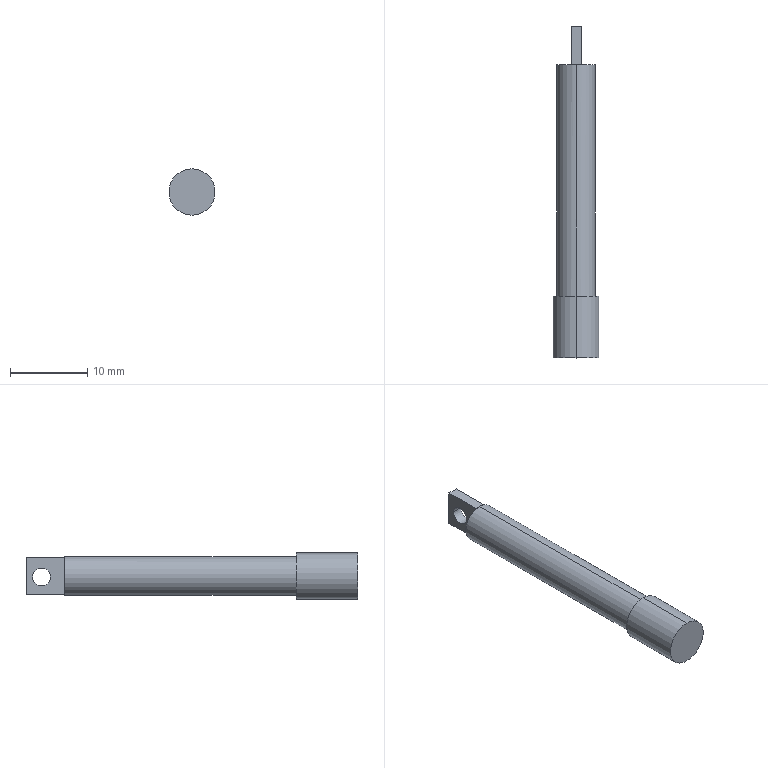Component | SolidWorks | Part22-2 | 1 solid | 17 faces | box 6 x 43 x 6 mm | volume 841 mm3 | plane 11 | cylinder 6 | commonest cylinder face diameters 2.308 x2 6 x2 5 x2
STEP:
#1=CARTESIAN_POINT('',(-6.067,11.196,-16.243));
#2=VERTEX_POINT('',#1);
#3=CARTESIAN_POINT('',(-6.067,11.105,-16.243));
#4=VERTEX_POINT('',#3);
#5=CARTESIAN_POINT('',(-6.067,11.15,-16.243));
#6=DIRECTION('',(1.,0.,0.));
#7=DIRECTION('',(0.,-1.,0.));
#8=AXIS2_PLACEMENT_3D('',#5,#6,#7);
#9=CIRCLE('',#8,0.04543);
#10=EDGE_CURVE('',#2,#4,#9,.T.);
#11=ORIENTED_EDGE('',*,*,#10,.F.);
#12=CARTESIAN_POINT('',(-6.016,11.196,-16.243));
#13=VERTEX_POINT('',#12);
#14=CARTESIAN_POINT('',(-6.212,11.196,-16.243));
#15=DIRECTION('',(1.,0.,0.));
#16=VECTOR('',#15,39.37);
#17=LINE('',#14,#16);
#18=EDGE_CURVE('',#2,#13,#17,.T.);
#19=ORIENTED_EDGE('',*,*,#18,.T.);
#20=CARTESIAN_POINT('',(-6.016,11.105,-16.243));
#21=VERTEX_POINT('',#20);
#22=CARTESIAN_POINT('',(-6.016,11.15,-16.243));
#23=DIRECTION('',(1.,0.,0.));
#24=DIRECTION('',(0.,-1.,0.));
#25=AXIS2_PLACEMENT_3D('',#22,#23,#24);
#26=CIRCLE('',#25,0.04543);
#27=EDGE_CURVE('',#13,#21,#26,.T.);
#28=ORIENTED_EDGE('',*,*,#27,.T.);
#29=CARTESIAN_POINT('',(-6.212,11.105,-16.243));
#30=DIRECTION('',(1.,0.,0.));
#31=VECTOR('',#30,39.37);
#32=LINE('',#29,#31);
#33=EDGE_CURVE('',#4,#21,#32,.T.);
#34=ORIENTED_EDGE('',*,*,#33,.F.);
#35=EDGE_LOOP('',(#11,#19,#28,#34));
#36=FACE_OUTER_BOUND('',#35,.T.);
#37=CARTESIAN_POINT('',(-6.212,11.15,-16.243));
#38=DIRECTION('',(1.,0.,0.));
#39=DIRECTION('',(0.,-1.,0.));
#40=AXIS2_PLACEMENT_3D('',#37,#38,#39);
#41=CYLINDRICAL_SURFACE('',#40,0.04543);
#42=ADVANCED_FACE('',(#36),#41,.F.);
#43=CARTESIAN_POINT('',(-6.044,9.537,-16.119));
#44=VERTEX_POINT('',#43);
#45=CARTESIAN_POINT('',(-6.044,9.537,-16.356));
#46=VERTEX_POINT('',#45);
#47=CARTESIAN_POINT('',(-6.044,9.537,-16.238));
#48=DIRECTION('',(0.,-1.,-0.));
#49=DIRECTION('',(0.,0.,1.));
#50=AXIS2_PLACEMENT_3D('',#47,#48,#49);
#51=CIRCLE('',#50,0.1181);
#52=EDGE_CURVE('',#44,#46,#51,.T.);
#53=ORIENTED_EDGE('',*,*,#52,.F.);
#54=CARTESIAN_POINT('',(-6.044,9.852,-16.119));
#55=VERTEX_POINT('',#54);
#56=CARTESIAN_POINT('',(-6.044,9.537,-16.119));
#57=DIRECTION('',(-0.,1.,0.));
#58=VECTOR('',#57,39.37);
#59=LINE('',#56,#58);
#60=EDGE_CURVE('',#44,#55,#59,.T.);
#61=ORIENTED_EDGE('',*,*,#60,.T.);
#62=CARTESIAN_POINT('',(-6.044,9.852,-16.356));
#63=VERTEX_POINT('',#62);
#64=CARTESIAN_POINT('',(-6.044,9.852,-16.238));
#65=DIRECTION('',(0.,-1.,-0.));
#66=DIRECTION('',(0.,0.,1.));
#67=AXIS2_PLACEMENT_3D('',#64,#65,#66);
#68=CIRCLE('',#67,0.1181);
#69=EDGE_CURVE('',#55,#63,#68,.T.);
#70=ORIENTED_EDGE('',*,*,#69,.T.);
#71=CARTESIAN_POINT('',(-6.044,9.537,-16.356));
#72=DIRECTION('',(-0.,1.,0.));
#73=VECTOR('',#72,39.37);
#74=LINE('',#71,#73);
#75=EDGE_CURVE('',#46,#63,#74,.T.);
#76=ORIENTED_EDGE('',*,*,#75,.F.);
#77=EDGE_LOOP('',(#53,#61,#70,#76));
#78=FACE_OUTER_BOUND('',#77,.T.);
#79=CARTESIAN_POINT('',(-6.044,9.537,-16.238));
#80=DIRECTION('',(-0.,1.,0.));
#81=DIRECTION('',(0.,0.,-1.));
#82=AXIS2_PLACEMENT_3D('',#79,#80,#81);
#83=CYLINDRICAL_SURFACE('',#82,0.1181);
#84=ADVANCED_FACE('',(#78),#83,.T.);
#85=CARTESIAN_POINT('',(-6.044,11.033,-16.336));
#86=VERTEX_POINT('',#85);
#87=CARTESIAN_POINT('',(-6.067,11.033,-16.142));
#88=VERTEX_POINT('',#87);
#89=CARTESIAN_POINT('',(-6.044,11.033,-16.238));
#90=DIRECTION('',(-0.,1.,0.));
#91=DIRECTION('',(0.,0.,-1.));
#92=AXIS2_PLACEMENT_3D('',#89,#90,#91);
#93=CIRCLE('',#92,0.09843);
#94=EDGE_CURVE('',#86,#88,#93,.T.);
#95=ORIENTED_EDGE('',*,*,#94,.F.);
#96=CARTESIAN_POINT('',(-6.044,9.852,-16.336));
#97=VERTEX_POINT('',#96);
#98=CARTESIAN_POINT('',(-6.044,11.033,-16.336));
#99=DIRECTION('',(0.,-1.,-0.));
#100=VECTOR('',#99,39.37);
#101=LINE('',#98,#100);
#102=EDGE_CURVE('',#86,#97,#101,.T.);
#103=ORIENTED_EDGE('',*,*,#102,.T.);
#104=CARTESIAN_POINT('',(-6.044,9.852,-16.139));
#105=VERTEX_POINT('',#104);
#106=CARTESIAN_POINT('',(-6.044,9.852,-16.238));
#107=DIRECTION('',(-0.,1.,0.));
#108=DIRECTION('',(0.,0.,-1.));
#109=AXIS2_PLACEMENT_3D('',#106,#107,#108);
#110=CIRCLE('',#109,0.09843);
#111=EDGE_CURVE('',#97,#105,#110,.T.);
#112=ORIENTED_EDGE('',*,*,#111,.T.);
#113=CARTESIAN_POINT('',(-6.044,11.033,-16.139));
#114=VERTEX_POINT('',#113);
#115=CARTESIAN_POINT('',(-6.044,11.033,-16.139));
#116=DIRECTION('',(0.,-1.,-0.));
#117=VECTOR('',#116,39.37);
#118=LINE('',#115,#117);
#119=EDGE_CURVE('',#114,#105,#118,.T.);
#120=ORIENTED_EDGE('',*,*,#119,.F.);
#121=CARTESIAN_POINT('',(-6.044,11.033,-16.238));
#122=DIRECTION('',(-0.,1.,0.));
#123=DIRECTION('',(0.,0.,-1.));
#124=AXIS2_PLACEMENT_3D('',#121,#122,#123);
#125=CIRCLE('',#124,0.09843);
#126=EDGE_CURVE('',#88,#114,#125,.T.);
#127=ORIENTED_EDGE('',*,*,#126,.F.);
#128=EDGE_LOOP('',(#95,#103,#112,#120,#127));
#129=FACE_OUTER_BOUND('',#128,.T.);
#130=CARTESIAN_POINT('',(-6.044,11.033,-16.238));
#131=DIRECTION('',(0.,-1.,-0.));
#132=DIRECTION('',(0.,0.,1.));
#133=AXIS2_PLACEMENT_3D('',#130,#131,#132);
#134=CYLINDRICAL_SURFACE('',#133,0.09843);
#135=ADVANCED_FACE('',(#129),#134,.T.);
#136=CARTESIAN_POINT('',(-6.021,11.033,-16.142));
#137=VERTEX_POINT('',#136);
#138=CARTESIAN_POINT('',(-6.067,11.033,-16.142));
#139=DIRECTION('',(1.,0.,0.));
#140=VECTOR('',#139,39.37);
#141=LINE('',#138,#140);
#142=EDGE_CURVE('',#88,#137,#141,.T.);
#143=ORIENTED_EDGE('',*,*,#142,.F.);
#144=ORIENTED_EDGE('',*,*,#126,.T.);
#145=CARTESIAN_POINT('',(-6.044,11.033,-16.238));
#146=DIRECTION('',(-0.,1.,0.));
#147=DIRECTION('',(0.,0.,-1.));
#148=AXIS2_PLACEMENT_3D('',#145,#146,#147);
#149=CIRCLE('',#148,0.09843);
#150=EDGE_CURVE('',#114,#137,#149,.T.);
#151=ORIENTED_EDGE('',*,*,#150,.T.);
#152=EDGE_LOOP('',(#143,#144,#151));
#153=FACE_OUTER_BOUND('',#152,.T.);
#154=CARTESIAN_POINT('',(-6.044,11.033,-16.238));
#155=DIRECTION('',(-0.,1.,0.));
#156=DIRECTION('',(0.,0.,-1.));
#157=AXIS2_PLACEMENT_3D('',#154,#155,#156);
#158=PLANE('',#157);
#159=ADVANCED_FACE('',(#153),#158,.T.);
#160=CARTESIAN_POINT('',(-6.067,11.033,-16.332));
#161=VERTEX_POINT('',#160);
#162=CARTESIAN_POINT('',(-6.067,11.033,-16.142));
#163=DIRECTION('',(0.,-0.,1.));
#164=VECTOR('',#163,39.37);
#165=LINE('',#162,#164);
#166=EDGE_CURVE('',#161,#88,#165,.T.);
#167=ORIENTED_EDGE('',*,*,#166,.F.);
#168=CARTESIAN_POINT('',(-6.016,11.033,-16.332));
#169=VERTEX_POINT('',#168);
#170=CARTESIAN_POINT('',(-6.067,11.033,-16.332));
#171=DIRECTION('',(-1.,-0.,-0.));
#172=VECTOR('',#171,39.37);
#173=LINE('',#170,#172);
#174=EDGE_CURVE('',#169,#161,#173,.T.);
#175=ORIENTED_EDGE('',*,*,#174,.F.);
#176=CARTESIAN_POINT('',(-6.044,11.033,-16.238));
#177=DIRECTION('',(-0.,1.,0.));
#178=DIRECTION('',(0.,0.,-1.));
#179=AXIS2_PLACEMENT_3D('',#176,#177,#178);
#180=CIRCLE('',#179,0.09843);
#181=EDGE_CURVE('',#169,#86,#180,.T.);
#182=ORIENTED_EDGE('',*,*,#181,.T.);
#183=ORIENTED_EDGE('',*,*,#94,.T.);
#184=EDGE_LOOP('',(#167,#175,#182,#183));
#185=FACE_OUTER_BOUND('',#184,.T.);
#186=CARTESIAN_POINT('',(-6.044,11.033,-16.238));
#187=DIRECTION('',(-0.,1.,0.));
#188=DIRECTION('',(0.,0.,-1.));
#189=AXIS2_PLACEMENT_3D('',#186,#187,#188);
#190=PLANE('',#189);
#191=ADVANCED_FACE('',(#185),#190,.T.);
#192=ORIENTED_EDGE('',*,*,#102,.F.);
#193=ORIENTED_EDGE('',*,*,#181,.F.);
#194=CARTESIAN_POINT('',(-6.016,11.033,-16.143));
#195=VERTEX_POINT('',#194);
#196=CARTESIAN_POINT('',(-6.044,11.033,-16.238));
#197=DIRECTION('',(-0.,1.,0.));
#198=DIRECTION('',(0.,0.,-1.));
#199=AXIS2_PLACEMENT_3D('',#196,#197,#198);
#200=CIRCLE('',#199,0.09843);
#201=EDGE_CURVE('',#195,#169,#200,.T.);
#202=ORIENTED_EDGE('',*,*,#201,.F.);
#203=CARTESIAN_POINT('',(-6.044,11.033,-16.238));
#204=DIRECTION('',(-0.,1.,0.));
#205=DIRECTION('',(0.,0.,-1.));
#206=AXIS2_PLACEMENT_3D('',#203,#204,#205);
#207=CIRCLE('',#206,0.09843);
#208=EDGE_CURVE('',#137,#195,#207,.T.);
#209=ORIENTED_EDGE('',*,*,#208,.F.);
#210=ORIENTED_EDGE('',*,*,#150,.F.);
#211=ORIENTED_EDGE('',*,*,#119,.T.);
#212=CARTESIAN_POINT('',(-6.044,9.852,-16.238));
#213=DIRECTION('',(-0.,1.,0.));
#214=DIRECTION('',(0.,0.,-1.));
#215=AXIS2_PLACEMENT_3D('',#212,#213,#214);
#216=CIRCLE('',#215,0.09843);
#217=EDGE_CURVE('',#105,#97,#216,.T.);
#218=ORIENTED_EDGE('',*,*,#217,.T.);
#219=EDGE_LOOP('',(#192,#193,#202,#209,#210,#211,#218));
#220=FACE_OUTER_BOUND('',#219,.T.);
#221=CARTESIAN_POINT('',(-6.044,11.033,-16.238));
#222=DIRECTION('',(0.,-1.,-0.));
#223=DIRECTION('',(0.,0.,1.));
#224=AXIS2_PLACEMENT_3D('',#221,#222,#223);
#225=CYLINDRICAL_SURFACE('',#224,0.09843);
#226=ADVANCED_FACE('',(#220),#225,.T.);
#227=CARTESIAN_POINT('',(-6.016,11.033,-16.142));
#228=DIRECTION('',(0.,0.,-1.));
#229=VECTOR('',#228,39.37);
#230=LINE('',#227,#229);
#231=EDGE_CURVE('',#195,#169,#230,.T.);
#232=ORIENTED_EDGE('',*,*,#231,.F.);
#233=ORIENTED_EDGE('',*,*,#201,.T.);
#234=EDGE_LOOP('',(#232,#233));
#235=FACE_OUTER_BOUND('',#234,.T.);
#236=CARTESIAN_POINT('',(-6.044,11.033,-16.238));
#237=DIRECTION('',(-0.,1.,0.));
#238=DIRECTION('',(0.,0.,-1.));
#239=AXIS2_PLACEMENT_3D('',#236,#237,#238);
#240=PLANE('',#239);
#241=ADVANCED_FACE('',(#235),#240,.T.);
#242=ORIENTED_EDGE('',*,*,#60,.F.);
#243=CARTESIAN_POINT('',(-6.044,9.537,-16.238));
#244=DIRECTION('',(0.,-1.,-0.));
#245=DIRECTION('',(0.,0.,1.));
#246=AXIS2_PLACEMENT_3D('',#243,#244,#245);
#247=CIRCLE('',#246,0.1181);
#248=EDGE_CURVE('',#46,#44,#247,.T.);
#249=ORIENTED_EDGE('',*,*,#248,.F.);
#250=ORIENTED_EDGE('',*,*,#75,.T.);
#251=CARTESIAN_POINT('',(-6.044,9.852,-16.238));
#252=DIRECTION('',(0.,-1.,-0.));
#253=DIRECTION('',(0.,0.,1.));
#254=AXIS2_PLACEMENT_3D('',#251,#252,#253);
#255=CIRCLE('',#254,0.1181);
#256=EDGE_CURVE('',#63,#55,#255,.T.);
#257=ORIENTED_EDGE('',*,*,#256,.T.);
#258=EDGE_LOOP('',(#242,#249,#250,#257));
#259=FACE_OUTER_BOUND('',#258,.T.);
#260=CARTESIAN_POINT('',(-6.044,9.537,-16.238));
#261=DIRECTION('',(-0.,1.,0.));
#262=DIRECTION('',(0.,0.,-1.));
#263=AXIS2_PLACEMENT_3D('',#260,#261,#262);
#264=CYLINDRICAL_SURFACE('',#263,0.1181);
#265=ADVANCED_FACE('',(#259),#264,.T.);
#266=ORIENTED_EDGE('',*,*,#248,.T.);
#267=ORIENTED_EDGE('',*,*,#52,.T.);
#268=EDGE_LOOP('',(#266,#267));
#269=FACE_OUTER_BOUND('',#268,.T.);
#270=CARTESIAN_POINT('',(-6.044,9.537,-16.238));
#271=DIRECTION('',(0.,-1.,-0.));
#272=DIRECTION('',(0.,-0.,1.));
#273=AXIS2_PLACEMENT_3D('',#270,#271,#272);
#274=PLANE('',#273);
#275=ADVANCED_FACE('',(#269),#274,.T.);
#276=ORIENTED_EDGE('',*,*,#217,.F.);
#277=ORIENTED_EDGE('',*,*,#111,.F.);
#278=EDGE_LOOP('',(#276,#277));
#279=FACE_BOUND('',#278,.T.);
#280=ORIENTED_EDGE('',*,*,#256,.F.);
#281=ORIENTED_EDGE('',*,*,#69,.F.);
#282=EDGE_LOOP('',(#280,#281));
#283=FACE_OUTER_BOUND('',#282,.T.);
#284=CARTESIAN_POINT('',(-6.044,9.852,-16.238));
#285=DIRECTION('',(0.,-1.,-0.));
#286=DIRECTION('',(0.,-0.,1.));
#287=AXIS2_PLACEMENT_3D('',#284,#285,#286);
#288=PLANE('',#287);
#289=ADVANCED_FACE('',(#279,#283),#288,.F.);
#290=CARTESIAN_POINT('',(-6.016,11.033,-16.142));
#291=VERTEX_POINT('',#290);
#292=CARTESIAN_POINT('',(-6.067,11.033,-16.142));
#293=DIRECTION('',(1.,0.,0.));
#294=VECTOR('',#293,39.37);
#295=LINE('',#292,#294);
#296=EDGE_CURVE('',#137,#291,#295,.T.);
#297=ORIENTED_EDGE('',*,*,#296,.F.);
#298=ORIENTED_EDGE('',*,*,#208,.T.);
#299=CARTESIAN_POINT('',(-6.016,11.033,-16.142));
#300=DIRECTION('',(0.,0.,-1.));
#301=VECTOR('',#300,39.37);
#302=LINE('',#299,#301);
#303=EDGE_CURVE('',#291,#195,#302,.T.);
#304=ORIENTED_EDGE('',*,*,#303,.F.);
#305=EDGE_LOOP('',(#297,#298,#304));
#306=FACE_OUTER_BOUND('',#305,.T.);
#307=CARTESIAN_POINT('',(4.488,11.033,-9.937));
#308=DIRECTION('',(-0.,1.,0.));
#309=DIRECTION('',(0.,0.,-1.));
#310=AXIS2_PLACEMENT_3D('',#307,#308,#309);
#311=PLANE('',#310);
#312=ADVANCED_FACE('',(#306),#311,.F.);
#313=ORIENTED_EDGE('',*,*,#142,.T.);
#314=ORIENTED_EDGE('',*,*,#296,.T.);
#315=CARTESIAN_POINT('',(-6.016,11.23,-16.142));
#316=VERTEX_POINT('',#315);
#317=CARTESIAN_POINT('',(-6.016,11.23,-16.142));
#318=DIRECTION('',(0.,-1.,-0.));
#319=VECTOR('',#318,39.37);
#320=LINE('',#317,#319);
#321=EDGE_CURVE('',#316,#291,#320,.T.);
#322=ORIENTED_EDGE('',*,*,#321,.F.);
#323=CARTESIAN_POINT('',(-6.067,11.23,-16.142));
#324=VERTEX_POINT('',#323);
#325=CARTESIAN_POINT('',(-6.067,11.23,-16.142));
#326=DIRECTION('',(1.,0.,0.));
#327=VECTOR('',#326,39.37);
#328=LINE('',#325,#327);
#329=EDGE_CURVE('',#324,#316,#328,.T.);
#330=ORIENTED_EDGE('',*,*,#329,.F.);
#331=CARTESIAN_POINT('',(-6.067,11.23,-16.142));
#332=DIRECTION('',(0.,-1.,-0.));
#333=VECTOR('',#332,39.37);
#334=LINE('',#331,#333);
#335=EDGE_CURVE('',#324,#88,#334,.T.);
#336=ORIENTED_EDGE('',*,*,#335,.T.);
#337=EDGE_LOOP('',(#313,#314,#322,#330,#336));
#338=FACE_OUTER_BOUND('',#337,.T.);
#339=CARTESIAN_POINT('',(-6.067,11.23,-16.142));
#340=DIRECTION('',(-0.,0.,-1.));
#341=DIRECTION('',(0.,-1.,-0.));
#342=AXIS2_PLACEMENT_3D('',#339,#340,#341);
#343=PLANE('',#342);
#344=ADVANCED_FACE('',(#338),#343,.F.);
#345=CARTESIAN_POINT('',(-6.016,11.15,-16.243));
#346=DIRECTION('',(1.,0.,0.));
#347=DIRECTION('',(0.,-1.,0.));
#348=AXIS2_PLACEMENT_3D('',#345,#346,#347);
#349=CIRCLE('',#348,0.04543);
#350=EDGE_CURVE('',#21,#13,#349,.T.);
#351=ORIENTED_EDGE('',*,*,#350,.F.);
#352=ORIENTED_EDGE('',*,*,#27,.F.);
#353=EDGE_LOOP('',(#351,#352));
#354=FACE_BOUND('',#353,.T.);
#355=ORIENTED_EDGE('',*,*,#303,.T.);
#356=ORIENTED_EDGE('',*,*,#231,.T.);
#357=CARTESIAN_POINT('',(-6.016,11.23,-16.332));
#358=VERTEX_POINT('',#357);
#359=CARTESIAN_POINT('',(-6.016,11.23,-16.332));
#360=DIRECTION('',(0.,-1.,-0.));
#361=VECTOR('',#360,39.37);
#362=LINE('',#359,#361);
#363=EDGE_CURVE('',#358,#169,#362,.T.);
#364=ORIENTED_EDGE('',*,*,#363,.F.);
#365=CARTESIAN_POINT('',(-6.016,11.23,-16.142));
#366=DIRECTION('',(0.,0.,-1.));
#367=VECTOR('',#366,39.37);
#368=LINE('',#365,#367);
#369=EDGE_CURVE('',#316,#358,#368,.T.);
#370=ORIENTED_EDGE('',*,*,#369,.F.);
#371=ORIENTED_EDGE('',*,*,#321,.T.);
#372=EDGE_LOOP('',(#355,#356,#364,#370,#371));
#373=FACE_OUTER_BOUND('',#372,.T.);
#374=CARTESIAN_POINT('',(-6.016,11.23,-16.142));
#375=DIRECTION('',(-1.,-0.,-0.));
#376=DIRECTION('',(-0.,1.,0.));
#377=AXIS2_PLACEMENT_3D('',#374,#375,#376);
#378=PLANE('',#377);
#379=ADVANCED_FACE('',(#354,#373),#378,.F.);
#380=ORIENTED_EDGE('',*,*,#174,.T.);
#381=CARTESIAN_POINT('',(-6.067,11.23,-16.332));
#382=VERTEX_POINT('',#381);
#383=CARTESIAN_POINT('',(-6.067,11.23,-16.332));
#384=DIRECTION('',(0.,-1.,-0.));
#385=VECTOR('',#384,39.37);
#386=LINE('',#383,#385);
#387=EDGE_CURVE('',#382,#161,#386,.T.);
#388=ORIENTED_EDGE('',*,*,#387,.F.);
#389=CARTESIAN_POINT('',(-6.067,11.23,-16.332));
#390=DIRECTION('',(-1.,-0.,-0.));
#391=VECTOR('',#390,39.37);
#392=LINE('',#389,#391);
#393=EDGE_CURVE('',#358,#382,#392,.T.);
#394=ORIENTED_EDGE('',*,*,#393,.F.);
#395=ORIENTED_EDGE('',*,*,#363,.T.);
#396=EDGE_LOOP('',(#380,#388,#394,#395));
#397=FACE_OUTER_BOUND('',#396,.T.);
#398=CARTESIAN_POINT('',(-6.067,11.23,-16.332));
#399=DIRECTION('',(0.,-0.,1.));
#400=DIRECTION('',(-0.,1.,0.));
#401=AXIS2_PLACEMENT_3D('',#398,#399,#400);
#402=PLANE('',#401);
#403=ADVANCED_FACE('',(#397),#402,.F.);
#404=CARTESIAN_POINT('',(-6.067,11.15,-16.243));
#405=DIRECTION('',(1.,0.,0.));
#406=DIRECTION('',(0.,-1.,0.));
#407=AXIS2_PLACEMENT_3D('',#404,#405,#406);
#408=CIRCLE('',#407,0.04543);
#409=EDGE_CURVE('',#4,#2,#408,.T.);
#410=ORIENTED_EDGE('',*,*,#409,.T.);
#411=ORIENTED_EDGE('',*,*,#10,.T.);
#412=EDGE_LOOP('',(#410,#411));
#413=FACE_BOUND('',#412,.T.);
#414=ORIENTED_EDGE('',*,*,#166,.T.);
#415=ORIENTED_EDGE('',*,*,#335,.F.);
#416=CARTESIAN_POINT('',(-6.067,11.23,-16.142));
#417=DIRECTION('',(0.,-0.,1.));
#418=VECTOR('',#417,39.37);
#419=LINE('',#416,#418);
#420=EDGE_CURVE('',#382,#324,#419,.T.);
#421=ORIENTED_EDGE('',*,*,#420,.F.);
#422=ORIENTED_EDGE('',*,*,#387,.T.);
#423=EDGE_LOOP('',(#414,#415,#421,#422));
#424=FACE_OUTER_BOUND('',#423,.T.);
#425=CARTESIAN_POINT('',(-6.067,11.23,-16.142));
#426=DIRECTION('',(1.,0.,0.));
#427=DIRECTION('',(0.,-1.,-0.));
#428=AXIS2_PLACEMENT_3D('',#425,#426,#427);
#429=PLANE('',#428);
#430=ADVANCED_FACE('',(#413,#424),#429,.F.);
#431=ORIENTED_EDGE('',*,*,#329,.T.);
#432=ORIENTED_EDGE('',*,*,#369,.T.);
#433=ORIENTED_EDGE('',*,*,#393,.T.);
#434=ORIENTED_EDGE('',*,*,#420,.T.);
#435=EDGE_LOOP('',(#431,#432,#433,#434));
#436=FACE_OUTER_BOUND('',#435,.T.);
#437=CARTESIAN_POINT('',(4.488,11.23,-9.937));
#438=DIRECTION('',(-0.,1.,0.));
#439=DIRECTION('',(0.,0.,-1.));
#440=AXIS2_PLACEMENT_3D('',#437,#438,#439);
#441=PLANE('',#440);
#442=ADVANCED_FACE('',(#436),#441,.T.);
#443=ORIENTED_EDGE('',*,*,#18,.F.);
#444=ORIENTED_EDGE('',*,*,#409,.F.);
#445=ORIENTED_EDGE('',*,*,#33,.T.);
#446=ORIENTED_EDGE('',*,*,#350,.T.);
#447=EDGE_LOOP('',(#443,#444,#445,#446));
#448=FACE_OUTER_BOUND('',#447,.T.);
#449=CARTESIAN_POINT('',(-6.212,11.15,-16.243));
#450=DIRECTION('',(1.,0.,0.));
#451=DIRECTION('',(0.,-1.,0.));
#452=AXIS2_PLACEMENT_3D('',#449,#450,#451);
#453=CYLINDRICAL_SURFACE('',#452,0.04543);
#454=ADVANCED_FACE('',(#448),#453,.F.);
#455=CLOSED_SHELL('',(#42,#84,#135,#159,#191,#226,#241,#265,#275,#289,#312,#344,#379,#403,#430,#442,#454));
#456=MANIFOLD_SOLID_BREP('',#455);
#457=CARTESIAN_POINT('',(0.,0.,0.));
#458=DIRECTION('',(0.,0.,1.));
#459=DIRECTION('',(1.,0.,0.));
#460=AXIS2_PLACEMENT_3D('',#457,#458,#459);
#461=(LENGTH_UNIT()NAMED_UNIT(*)SI_UNIT($,.METRE.));
#462=LENGTH_MEASURE_WITH_UNIT(LENGTH_MEASURE(0.0254),#461);
#463=DIMENSIONAL_EXPONENTS(1.,0.,0.,0.,0.,0.,0.);
#464=(CONVERSION_BASED_UNIT('',#462)LENGTH_UNIT()NAMED_UNIT(#463));
#465=UNCERTAINTY_MEASURE_WITH_UNIT(LENGTH_MEASURE(0.00001),#464,'','');
#466=(NAMED_UNIT(*)PLANE_ANGLE_UNIT()SI_UNIT($,.RADIAN.));
#467=(NAMED_UNIT(*)SI_UNIT($,.STERADIAN.)SOLID_ANGLE_UNIT());
#468=(GEOMETRIC_REPRESENTATION_CONTEXT(3)GLOBAL_UNCERTAINTY_ASSIGNED_CONTEXT((#465))GLOBAL_UNIT_ASSIGNED_CONTEXT((#464,#466,#467))REPRESENTATION_CONTEXT('',''));
#469=ADVANCED_BREP_SHAPE_REPRESENTATION('',(#456,#460),#468);
#470=COLOUR_RGB('',0.7922,0.8196,0.9333);
#471=FILL_AREA_STYLE_COLOUR('',#470);
#472=FILL_AREA_STYLE('',(#471));
#473=SURFACE_STYLE_FILL_AREA(#472);
#474=SURFACE_SIDE_STYLE('',(#473));
#475=SURFACE_STYLE_USAGE(.BOTH.,#474);
#476=PRESENTATION_STYLE_ASSIGNMENT((#475));
#477=STYLED_ITEM('',(#476),#456);
#478=(LENGTH_UNIT()NAMED_UNIT(*)SI_UNIT($,.METRE.));
#479=LENGTH_MEASURE_WITH_UNIT(LENGTH_MEASURE(0.0254),#478);
#480=DIMENSIONAL_EXPONENTS(1.,0.,0.,0.,0.,0.,0.);
#481=(CONVERSION_BASED_UNIT('',#479)LENGTH_UNIT()NAMED_UNIT(#480));
#482=UNCERTAINTY_MEASURE_WITH_UNIT(LENGTH_MEASURE(0.00001),#481,'','');
#483=(NAMED_UNIT(*)PLANE_ANGLE_UNIT()SI_UNIT($,.RADIAN.));
#484=(NAMED_UNIT(*)SI_UNIT($,.STERADIAN.)SOLID_ANGLE_UNIT());
#485=(GEOMETRIC_REPRESENTATION_CONTEXT(3)GLOBAL_UNCERTAINTY_ASSIGNED_CONTEXT((#482))GLOBAL_UNIT_ASSIGNED_CONTEXT((#481,#483,#484))REPRESENTATION_CONTEXT('',''));
#486=MECHANICAL_DESIGN_GEOMETRIC_PRESENTATION_REPRESENTATION('',(#477),#485);
#487=PRESENTATION_LAYER_ASSIGNMENT('','',(#477));